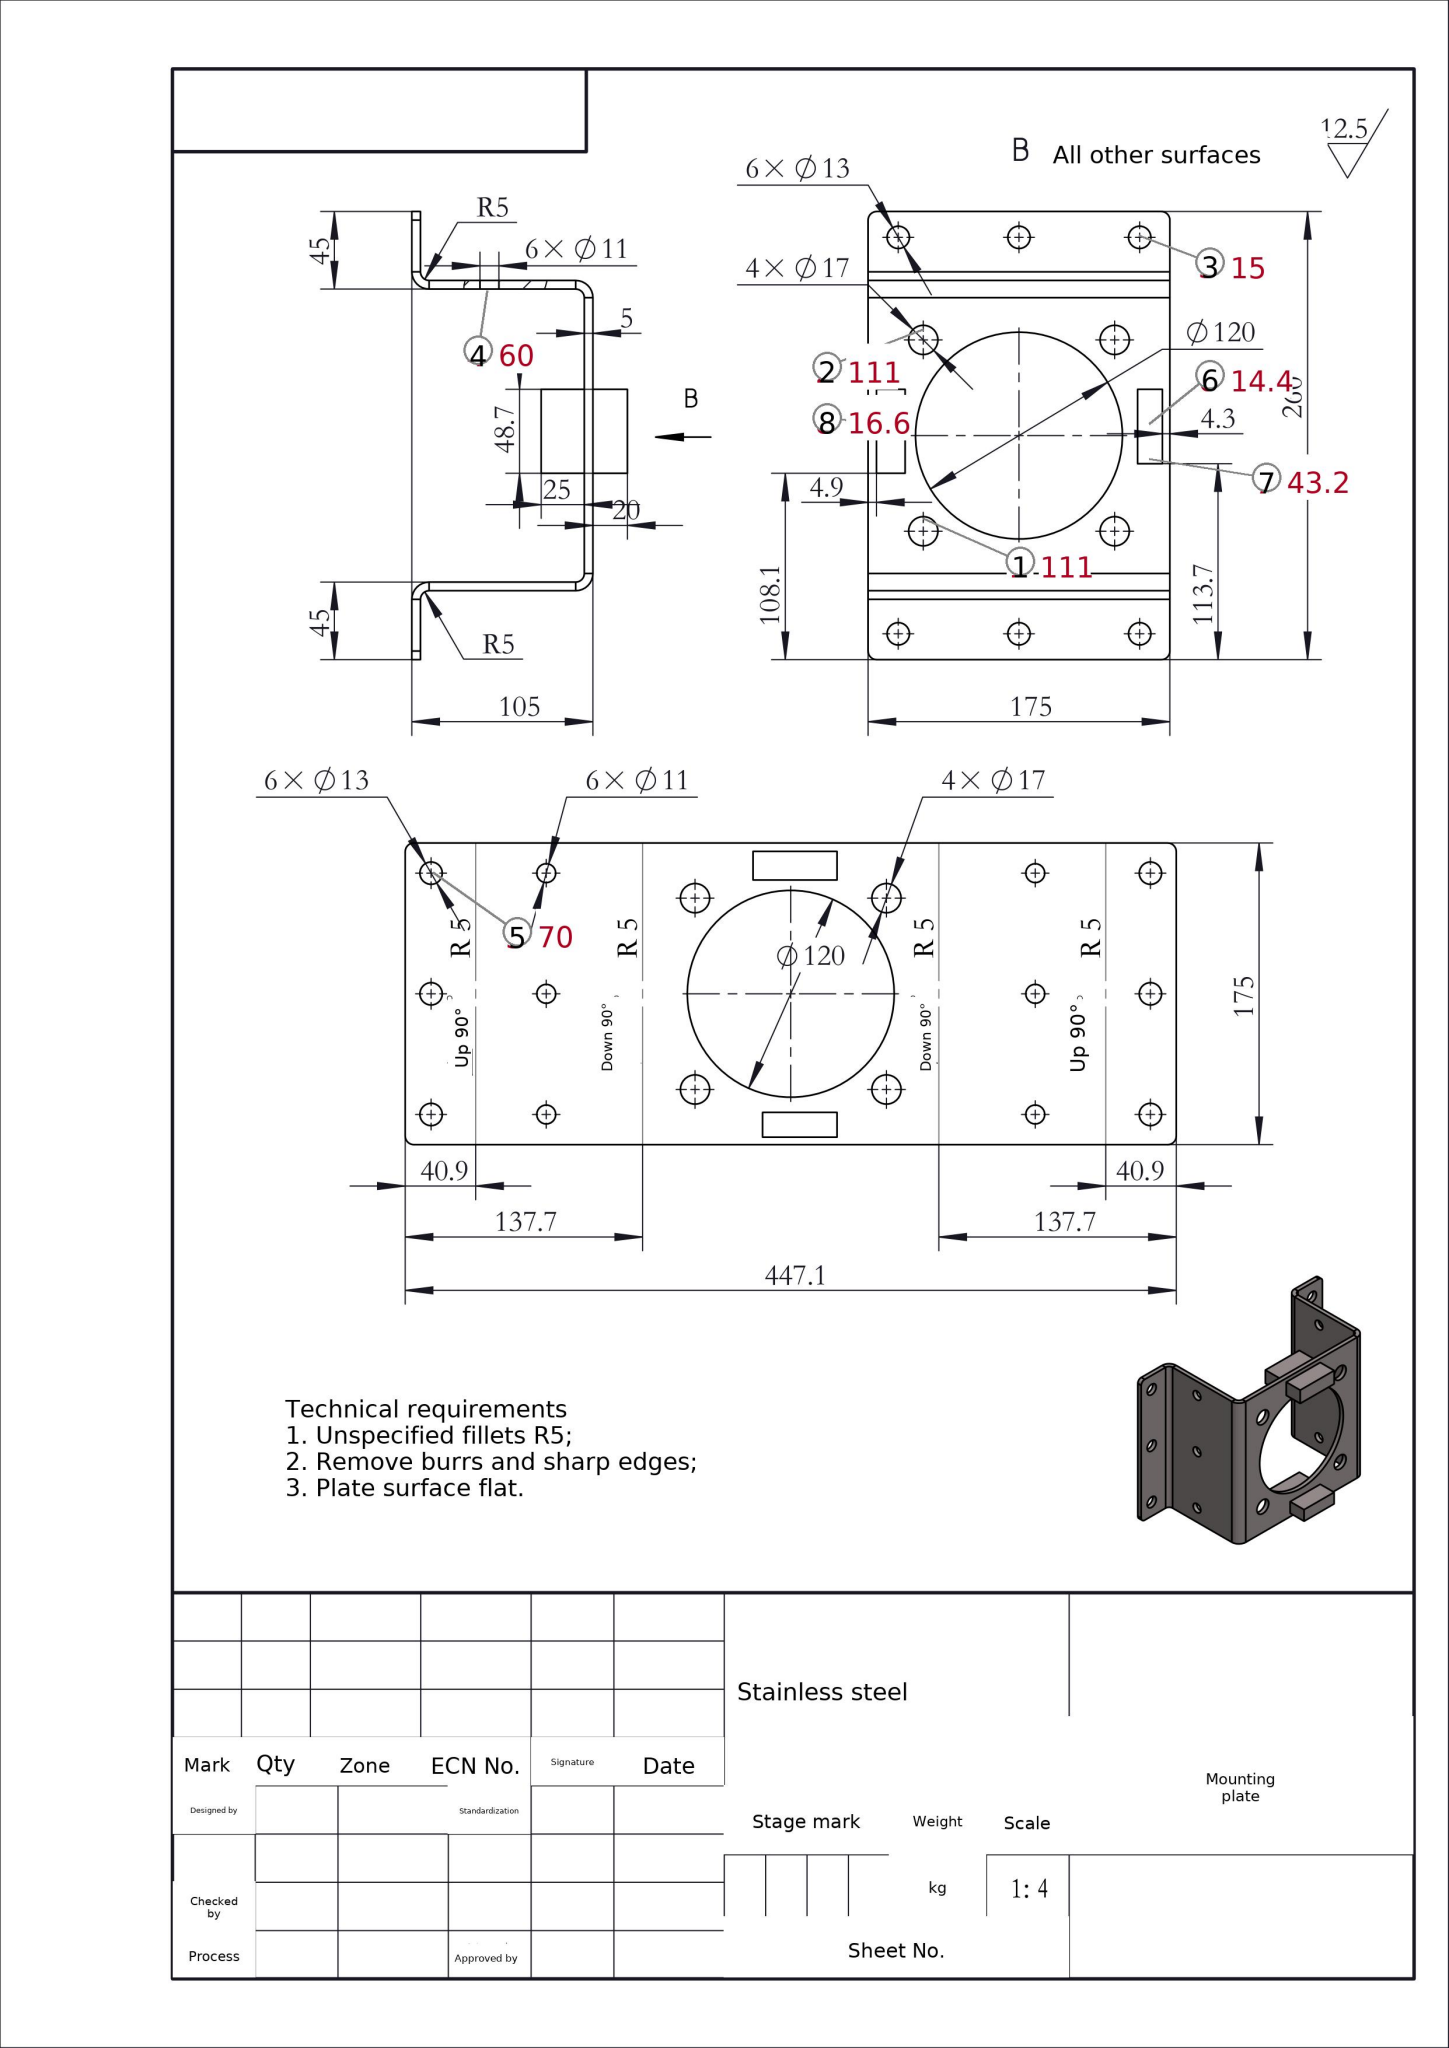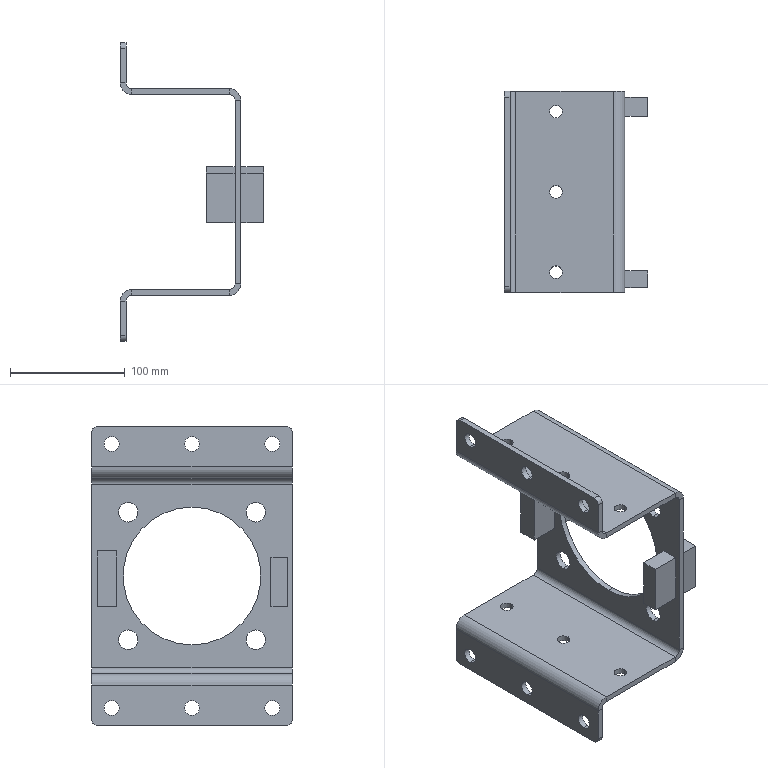Part | SolidWorks | mm | material Stainless steel | 1 solid | 96 faces | box 125 x 175 x 260 mm | volume 387569 mm3 | plane 50 | cylinder 46 | commonest cylinder face diameters 11 x12 13 x12 17 x8 10 x8 20 x4 120 x2